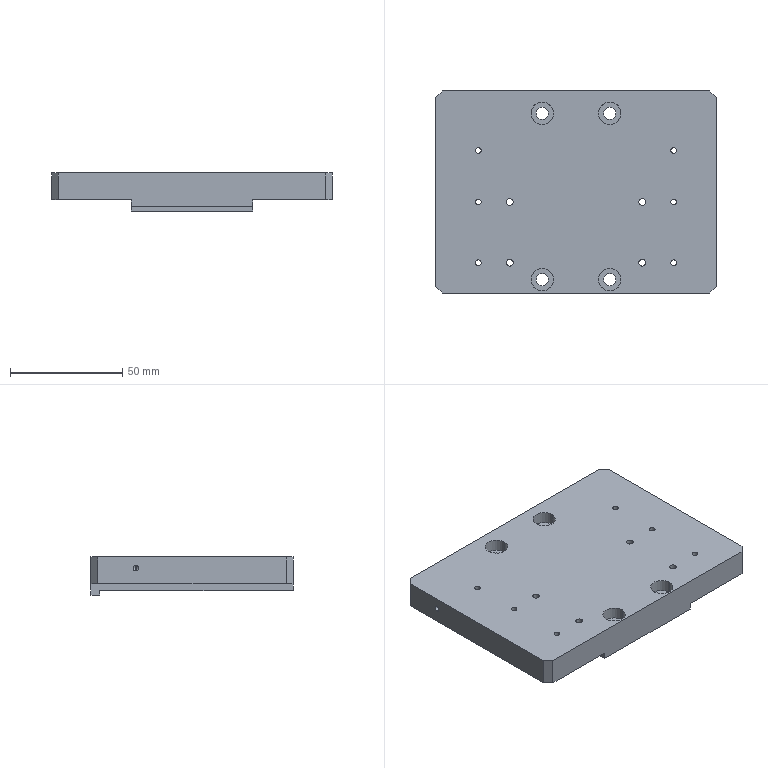Component | SolidWorks | SAWH02-03329A0MountingBase-1 | 1 solid | 80 faces | box 125 x 90 x 17 mm | volume 145708 mm3 | cylinder 48 | plane 20 | cone 12 | commonest cylinder face diameters 2.5 x16 4.2 x8 3 x8 10 x8 5.5 x8 | material 6061
build123d program:
from build123d import *

# Parameters (mm, degrees)
SKETCH1_W                                       = 125
SKETCH1_H                                       = 90
BOSS_EXTRUDE1_DEPTH                             = 17
SKETCH2_W                                       = 35.5
SKETCH2_H                                       = 90
CUT_EXTRUDE1_DEPTH                              = 5
M5_HEX_SOCKET_HEAD_CAP_SCREW_CBORE1_D           = 5.5
M5_HEX_SOCKET_HEAD_CAP_SCREW_CBORE1_CBORE_D     = 10
M5_HEX_SOCKET_HEAD_CAP_SCREW_CBORE1_CBORE_DEPTH = 5.4
SKETCH5_W                                       = 54
SKETCH5_H                                       = 86
CUT_EXTRUDE2_DEPTH                              = 2
M3_TAPPED_HOLE1_D                               = 2.5
SKETCH9_R                                       = 1.5
CUT_EXTRUDE3_DEPTH                              = 79.869
CHAMFER1_SIZE                                   = 3
M5_TAPPED_HOLE1_AT_2_COUNT                      = 2
M5_TAPPED_HOLE1_AT_2_PITCH                      = 16


with BuildPart() as part:
    # Sketch1 → Boss-Extrude1 (new body)
    with BuildSketch(Plane.XY):
        Rectangle(SKETCH1_W, SKETCH1_H)
    extrude(amount=BOSS_EXTRUDE1_DEPTH)

    # Sketch2 → Cut-Extrude1 (cut)
    with BuildSketch(Plane(origin=(0, 0, 0), x_dir=(-1, 0, 0), z_dir=(0, 0, -1))):
        with Locations((-44.75, 0)):
            Rectangle(SKETCH2_W, SKETCH2_H)
        with Locations((44.75, 0)):
            Rectangle(SKETCH2_W, SKETCH2_H)
    extrude(amount=-CUT_EXTRUDE1_DEPTH, mode=Mode.SUBTRACT)

    # M5 Hex Socket Head Cap Screw CBORE1 (through all)
    with Locations(Plane.XY.offset(17)):
        with Locations((-15, 35), (15, 35), (15, -39), (-15, -39)):
            CounterBoreHole(M5_HEX_SOCKET_HEAD_CAP_SCREW_CBORE1_D / 2, M5_HEX_SOCKET_HEAD_CAP_SCREW_CBORE1_CBORE_D / 2, M5_HEX_SOCKET_HEAD_CAP_SCREW_CBORE1_CBORE_DEPTH)

    # Sketch5 → Cut-Extrude2 (cut)
    with BuildSketch(Plane(origin=(0, 0, 0), x_dir=(-1, 0, 0), z_dir=(0, 0, -1))):
        with Locations((0, -2)):
            Rectangle(SKETCH5_W, SKETCH5_H)
    extrude(amount=-CUT_EXTRUDE2_DEPTH, mode=Mode.SUBTRACT)

    # M3 Tapped Hole1 (through all)
    with Locations(Plane.XY.offset(17)):
        with Locations((-43.5, 18.5), (-43.5, -4.5), (-43.5, -31.5), (43.5, -31.5), (43.5, -4.5), (43.5, 18.5)):
            Hole(M3_TAPPED_HOLE1_D / 2)

    # Sketch9 → Cut-Extrude3 (cut, through all)
    with BuildSketch(Plane.XY.offset(17)):
        with Locations((-29.5, -31.5)):
            Circle(SKETCH9_R)
        with Locations((-29.5, -4.5)):
            Circle(SKETCH9_R)
        with Locations(Location((29.5, -4.5, 0), (0, 0, 180))):
            Circle(SKETCH9_R)
        with Locations(Location((29.5, -31.5, 0), (0, 0, 180))):
            Circle(SKETCH9_R)
    extrude(amount=-CUT_EXTRUDE3_DEPTH, mode=Mode.SUBTRACT)

    # Chamfer1
    chamfer1_edges = [part.edges().sort_by_distance(p)[0] for p in [
        (62.5, -45, 11),
        (-62.5, -45, 11),
        (-62.5, 45, 11),
        (62.5, 45, 11),
    ]]
    chamfer(chamfer1_edges, length=CHAMFER1_SIZE)

    # Sketch11 → M3 Tapped Hole2 (revolve, cut)
    with BuildSketch(Plane(origin=(-62.5, 25, 12), x_dir=(0, 0, 1), z_dir=(0, 1, 0))):
        Polygon((0, 0), (0, 8.251), (1.25, 7.5), (1.25, 0), align=None)
    m3_tapped_hole2 = revolve(axis=Axis((-68.85, 25, 12), (1, 0, 0)), mode=Mode.SUBTRACT)

    # Mirror1: M3 Tapped Hole2 across plane
    add(m3_tapped_hole2.mirror(Plane(origin=(0, 0, 0), x_dir=(0, 0, 1), z_dir=(1, 0, 0))), mode=Mode.SUBTRACT)

    # Sketch13 → M5 Tapped Hole1 (revolve, cut)
    with BuildSketch(Plane(origin=(53.5, 45, 11), x_dir=(0, 0, 1), z_dir=(1, 0, 0))):
        Polygon((0, 0), (0, 13.662), (2.1, 12.4), (2.1, 0), align=None)
    m5_tapped_hole1 = revolve(axis=Axis((53.5, 51.35, 11), (0, -1, 0)), mode=Mode.SUBTRACT)

    # M5 Tapped Hole1 at 2: M5 Tapped Hole1 ×2
    with Locations(*[(-i * M5_TAPPED_HOLE1_AT_2_PITCH, 0, 0) for i in range(1, M5_TAPPED_HOLE1_AT_2_COUNT)]):
        add(m5_tapped_hole1, mode=Mode.SUBTRACT)

    # Mirror2: M5 Tapped Hole1 across plane
    add(m5_tapped_hole1.mirror(Plane(origin=(0, 0, 0), x_dir=(0, 0, 1), z_dir=(1, 0, 0))), mode=Mode.SUBTRACT)

    # Mirror2 copy 1 sketch → Mirror2 copy 1 (revolve, cut)
    with BuildSketch(Plane(origin=(-37.5, 45, 11), x_dir=(0, 0, 1), z_dir=(-1, 0, 0))):
        Polygon((0, 0), (0, -13.662), (2.1, -12.4), (2.1, 0), align=None)
    revolve(axis=Axis((-37.5, 51.35, 11), (0, 1, 0)), mode=Mode.SUBTRACT)


solid = part.part